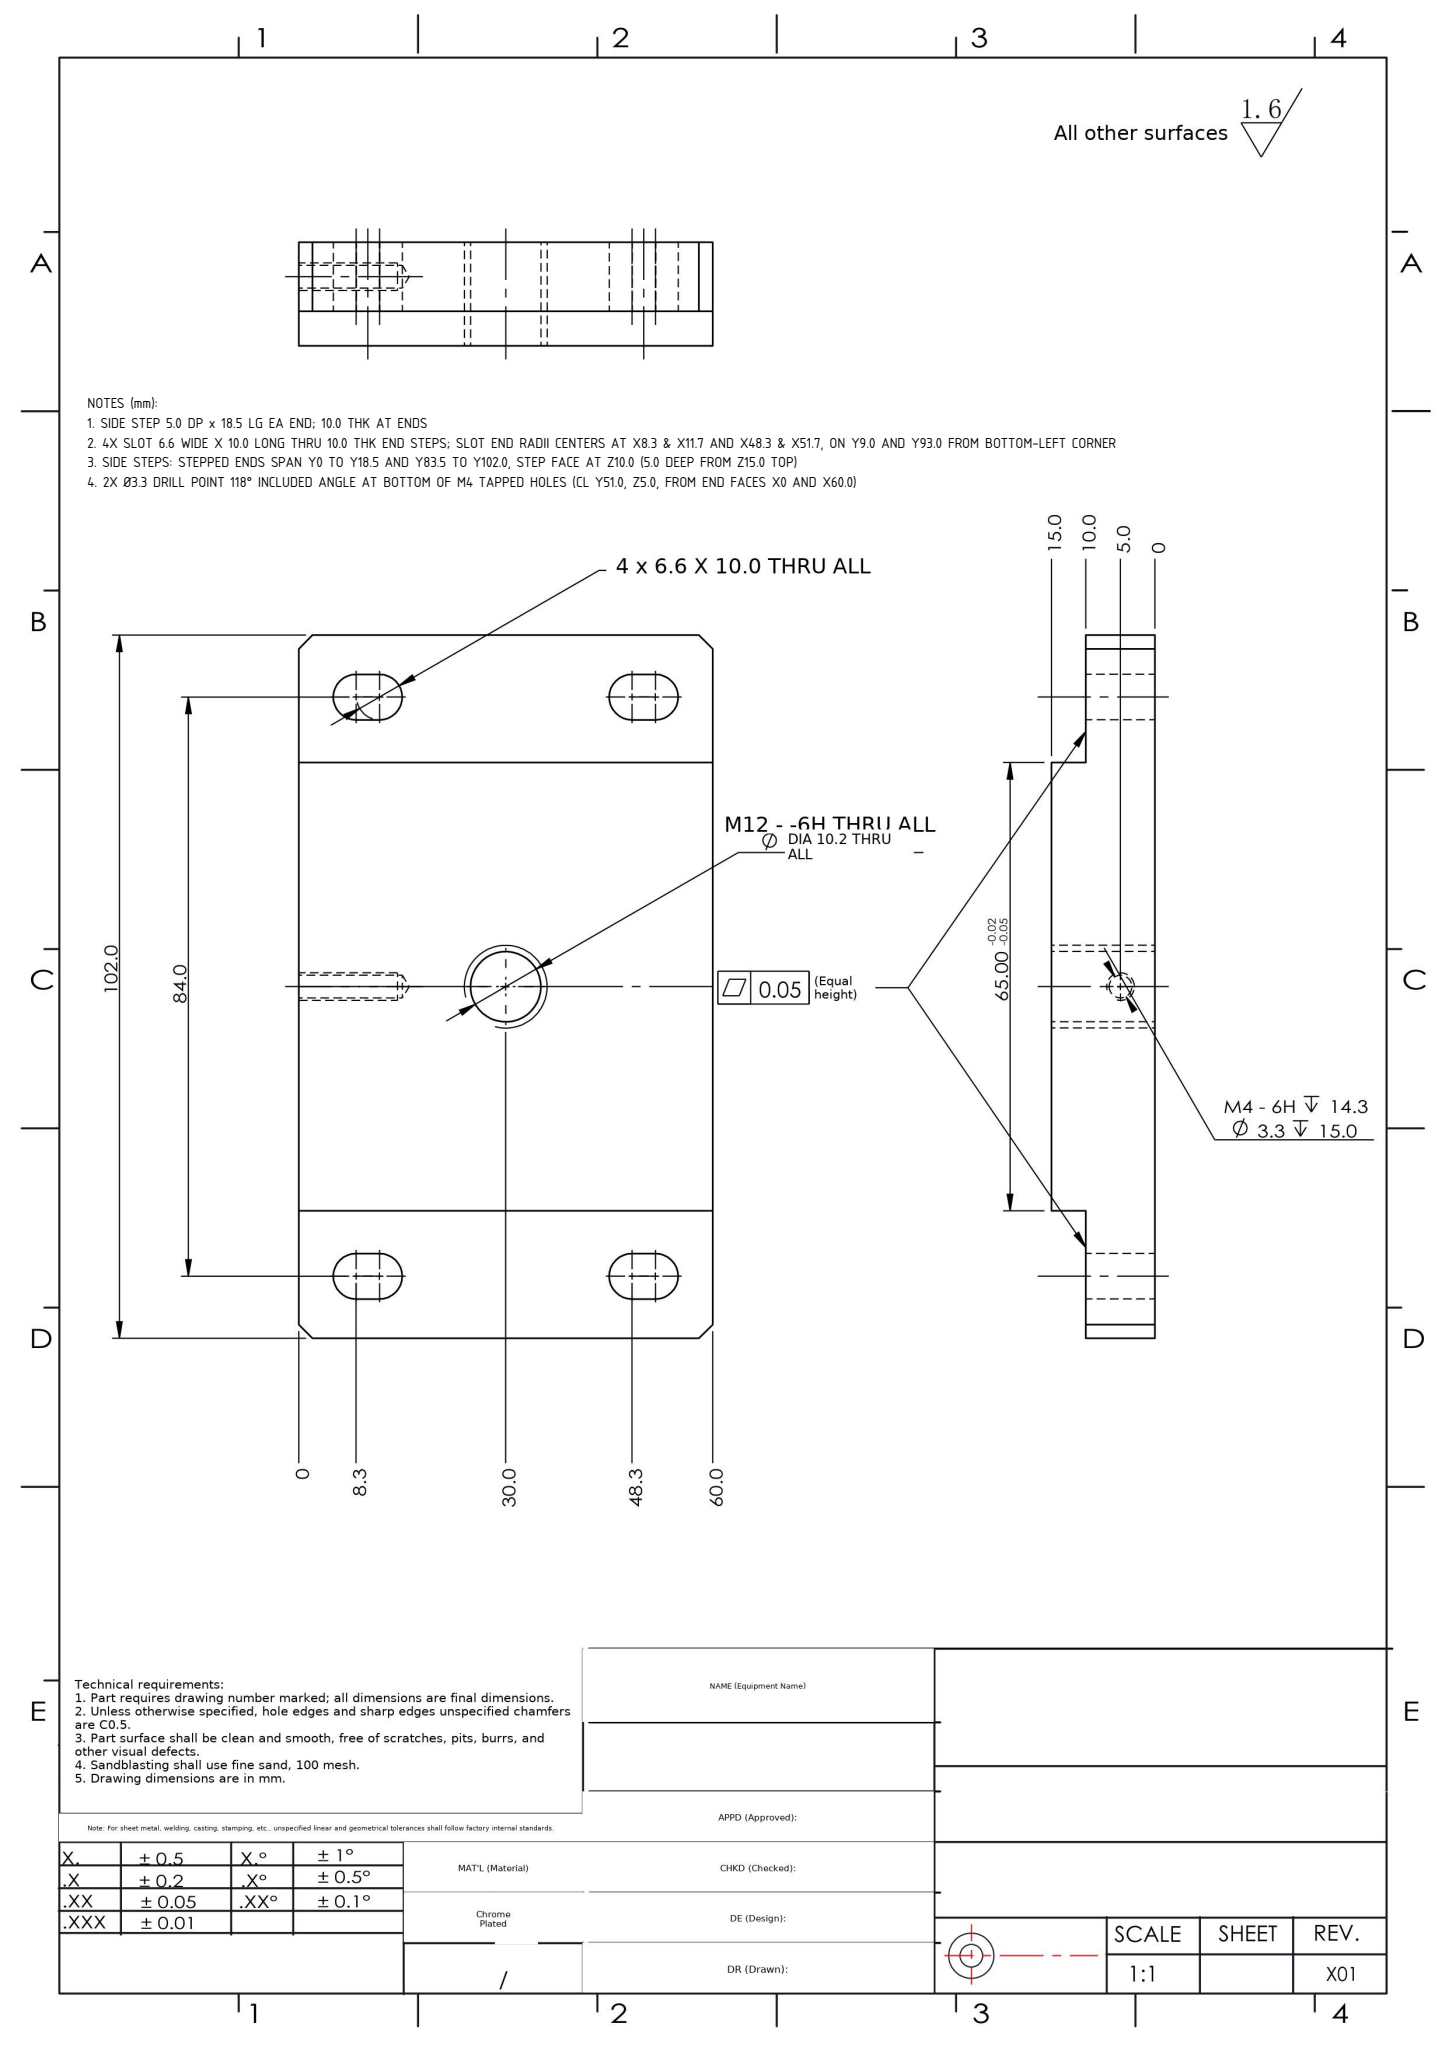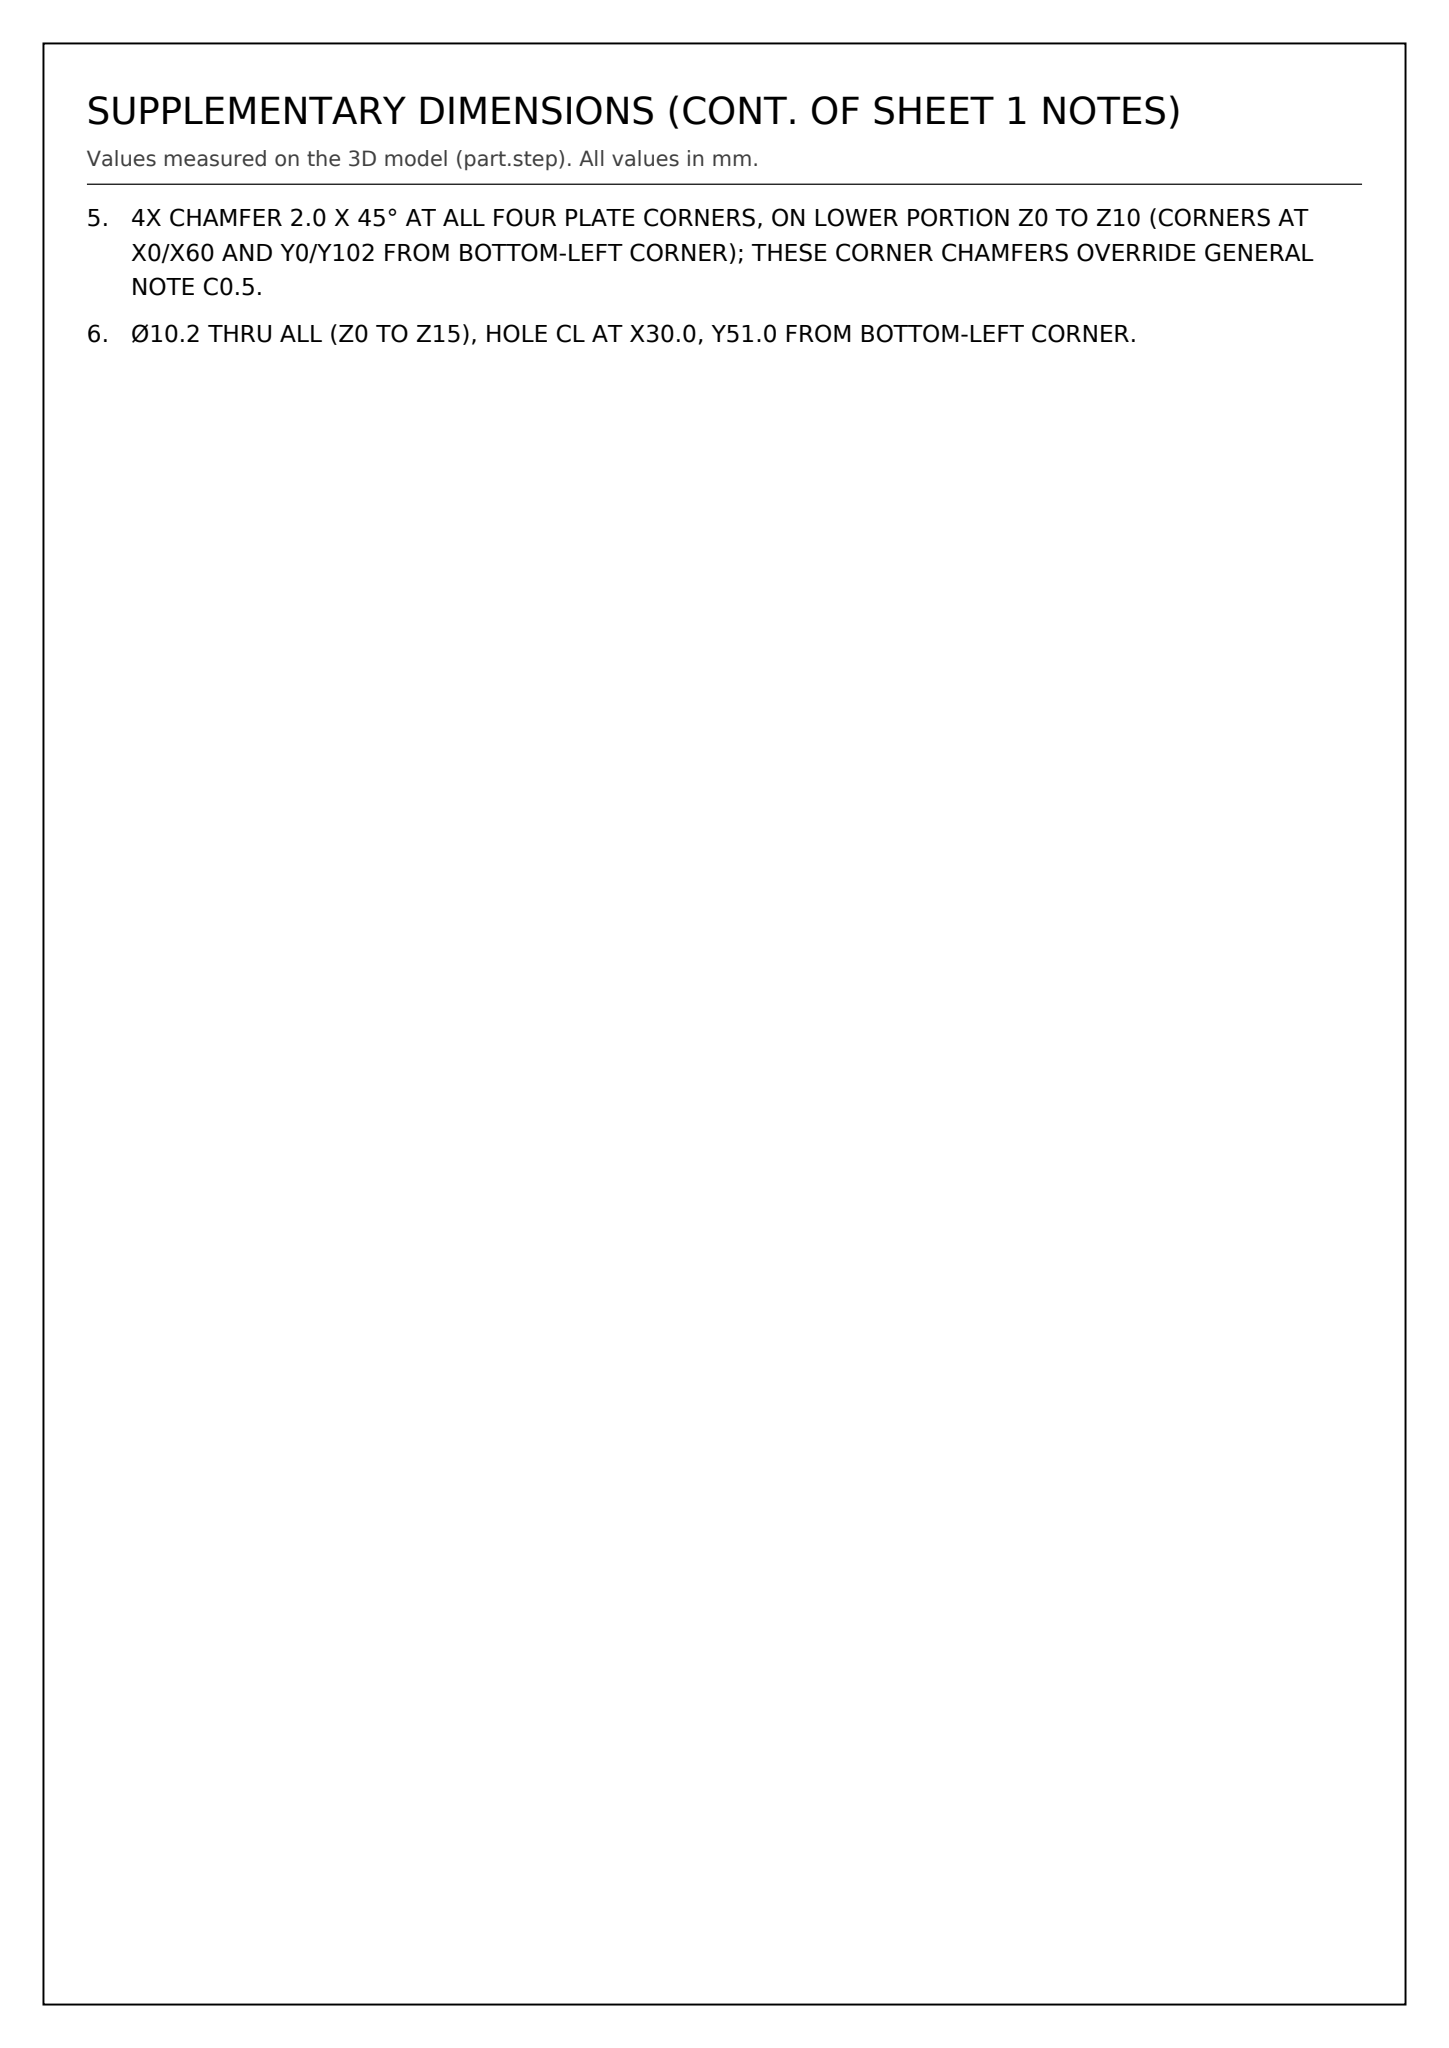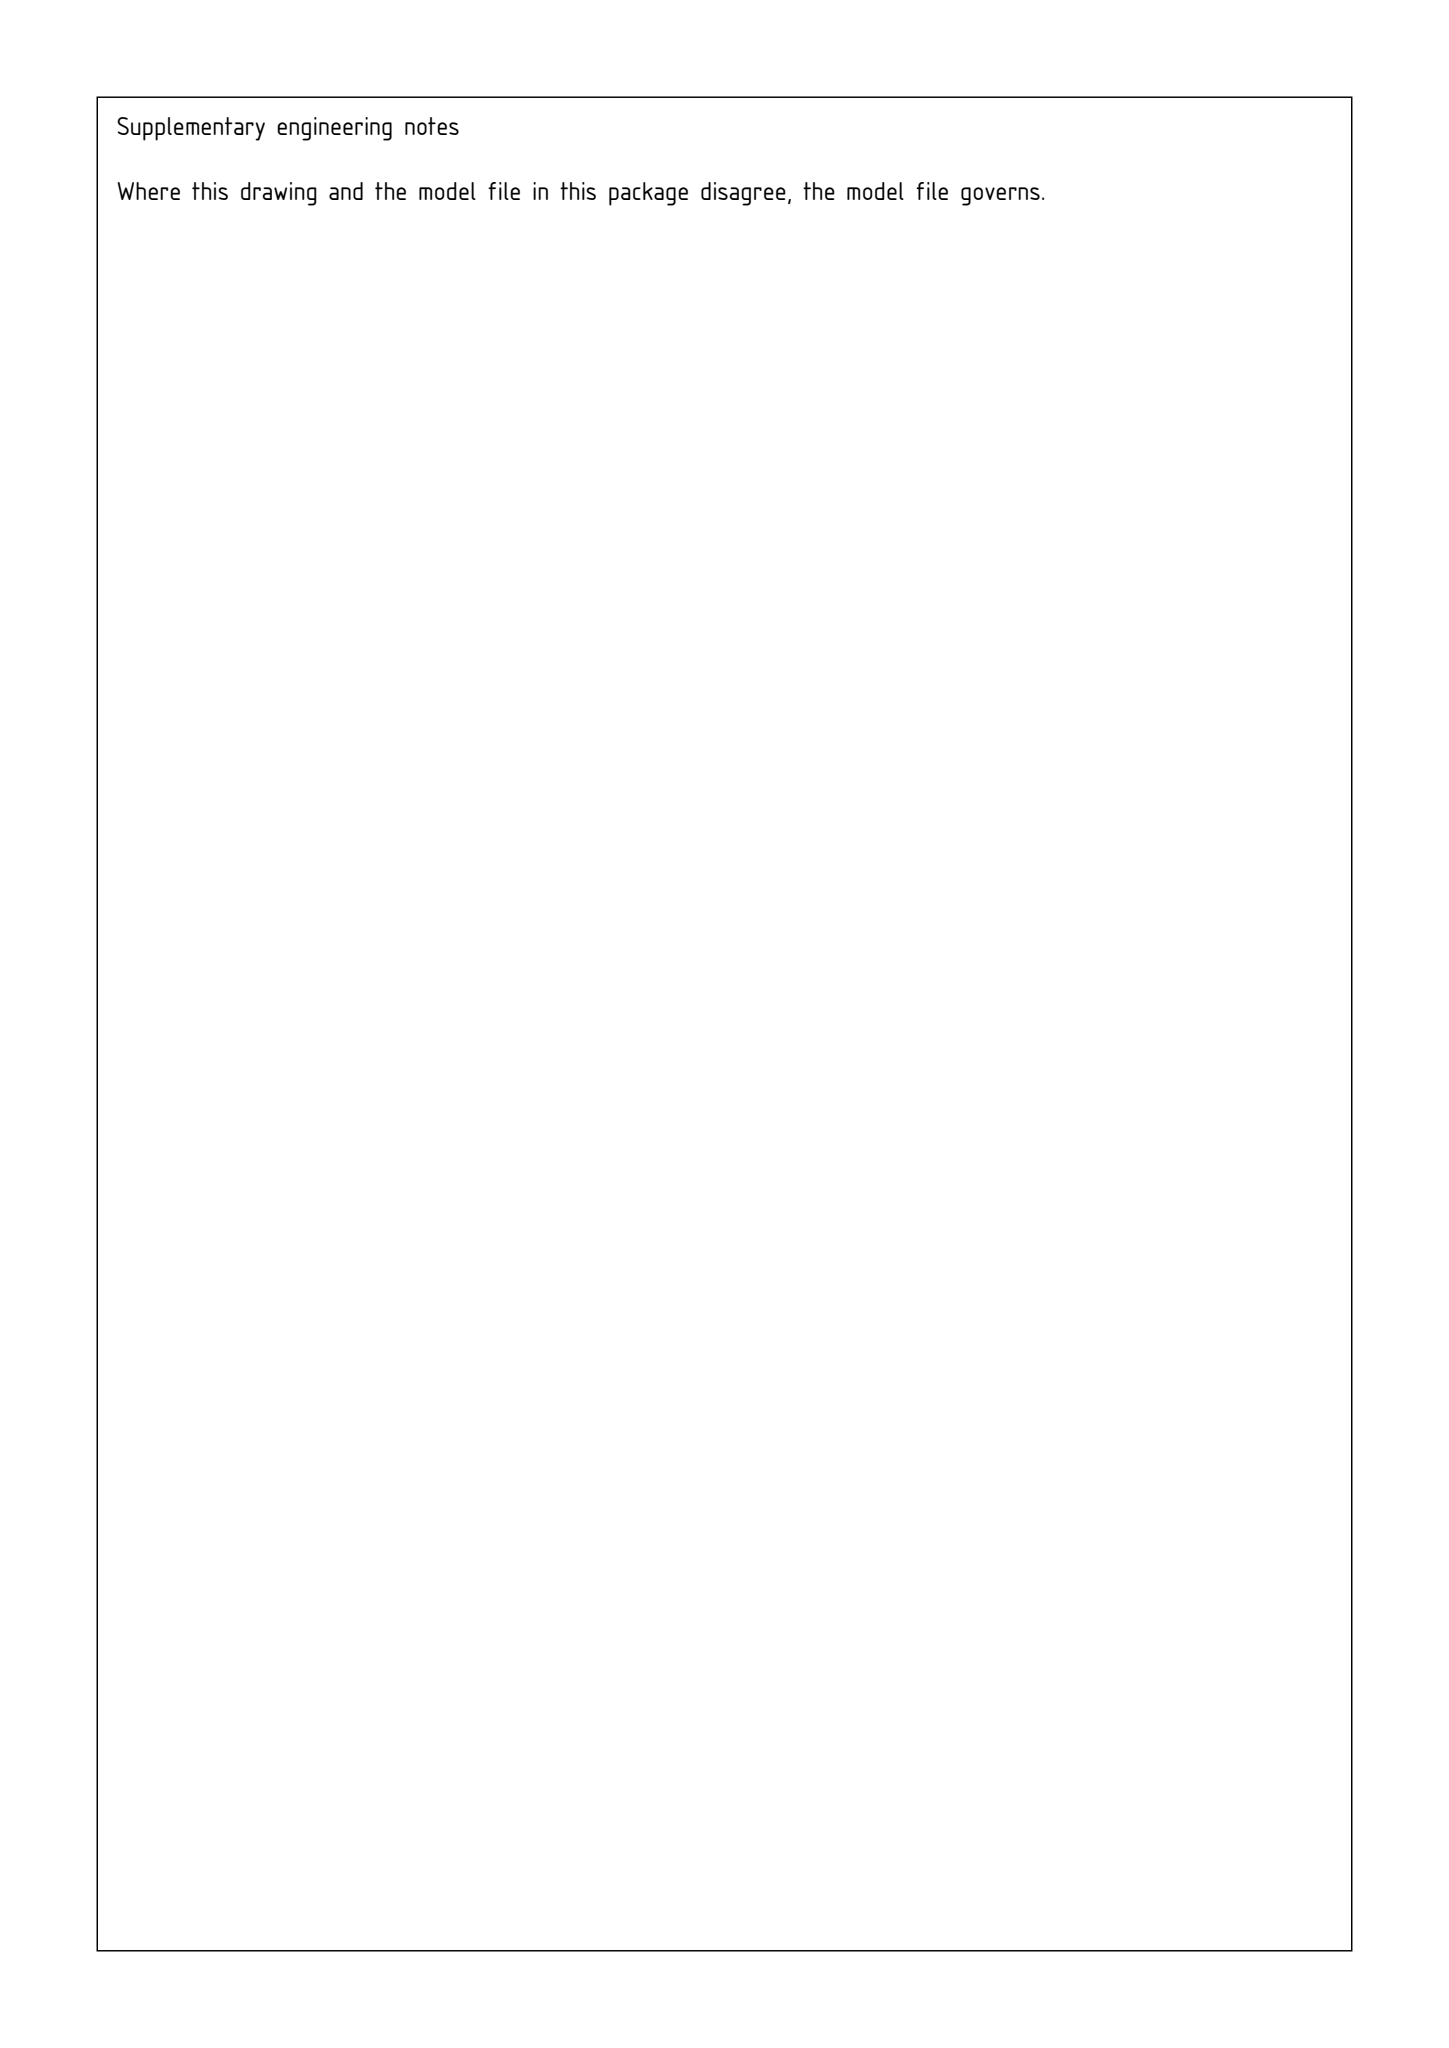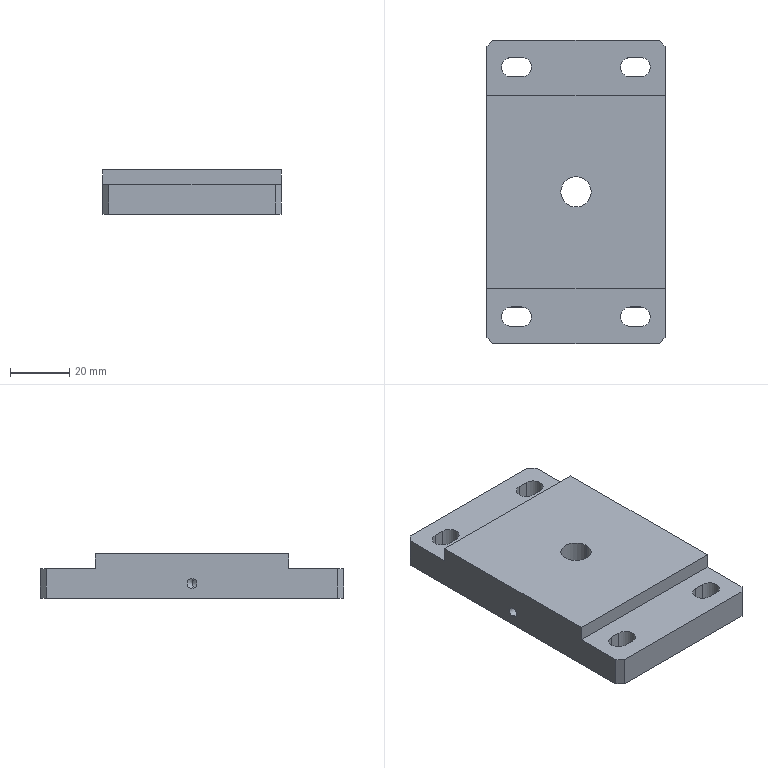Part | SolidWorks | mm | 1 solid | 40 faces | box 60 x 102 x 15 mm | volume 76997 mm3 | plane 22 | cylinder 16 | cone 2 | commonest cylinder face diameters 6.6 x12 10.2 x2 3.3 x2
Drawing notes:
SIDE STEP 5.0 DP x 18.5 LG EA END; 10.0 THK AT ENDS | from the solid: z-planes 0/10.0(2)/15.0 with y-planes 18.5 & 83.5; 83.5-18.5=65.00; 102.0-83.5=18.5
4X SLOT 6.6 WIDE X 10.0 LONG THRU 10.0 THK END STEPS; SLOT END RADII CENTERS AT X8.3 & X11.7 AND X48.3 & X51.7, ON Y9.0 AND Y93.0 FROM BOTTOM-LEFT CORNER | from the solid: cylinders 6.6 dia, axis z, length 10.0 at (8.3/11.7, 9.0) and (48.3/51.7, 9.0) and same at y93.0; planes y=5.7/12.3/89.7/96.3 (slot sides); plane z=10.0
SIDE STEPS: STEPPED ENDS SPAN Y0 TO Y18.5 AND Y83.5 TO Y102.0, STEP FACE AT Z10.0 (5.0 DEEP FROM Z15.0 TOP) | from the solid: axis_planes y=18.5, y=83.5, z=10.0, z=15.0; bbox 60.0 x 102.0 x 15.0
2X Ø3.3 DRILL POINT 118° INCLUDED ANGLE AT BOTTOM OF M4 TAPPED HOLES (CL Y51.0, Z5.0, FROM END FACES X0 AND X60.0) | from the solid: cones [118.0 included angle, ref_dia 3.3, count 2]; cylinders 3.3 dia, axis x, pos (y51.0, z5.0), length 15.0
4X CHAMFER 2.0 X 45° AT ALL FOUR PLATE CORNERS, ON LOWER PORTION Z0 TO Z10 (CORNERS AT X0/X60 AND Y0/Y102 FROM BOTTOM-LEFT CORNER); THESE CORNER CHAMFERS OVERRIDE GENERAL NOTE C0.5. | from the solid: inclined_planes: four 45°/45°/90° faces, size 2.0 x 2.0 x 10.0, bbox_from [0,0,0], [0,100,0], [58,0,0], [58,100,0]
Ø10.2 THRU ALL (Z0 TO Z15), HOLE CL AT X30.0, Y51.0 FROM BOTTOM-LEFT CORNER. | from the solid: cylinders: hole/bore dia 10.2, axis z at [30.0, 51.0], from 0.0 to 15.0, arc 360